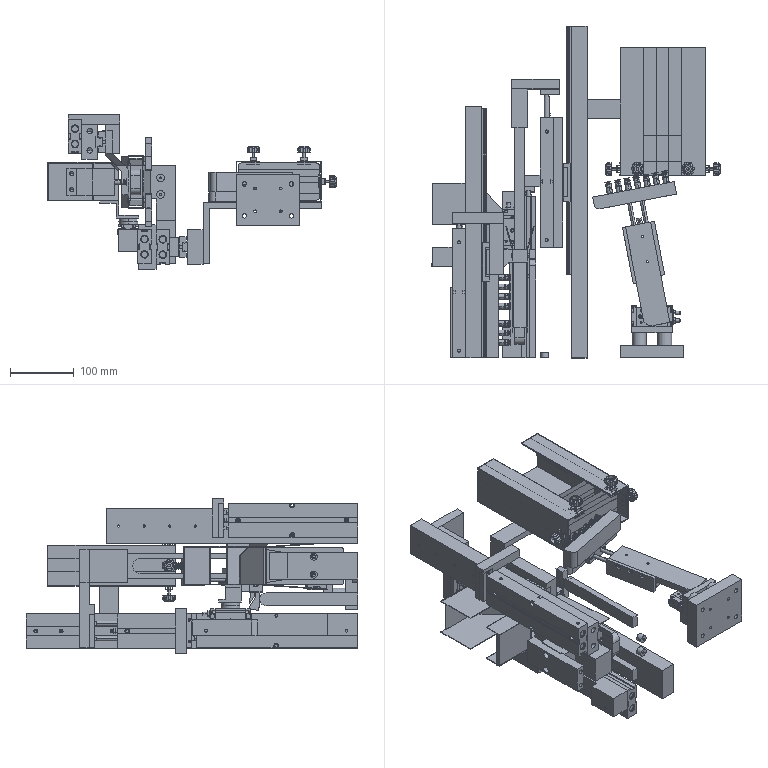Assembly | SolidWorks | mm | 91 component files | 107 solids | 3968 faces | box 451.44 x 520 x 242.54 mm | volume 3944049 mm3 | plane 1659 | cylinder 1465 | cone 700 | torus 144 | commonest cylinder face diameters 4.5 x136 6 x130 0.4 x90 8 x81 2.459 x80 4 x79 4.2 x70 3.5 x64
Bill of materials:
Counterweight | 2 |  | Rectangular prismatic block with a narrow slit running in from one top corner. The slit starts at an angle, turns straight along the length, and ends in a circular relief hole. A small cross hole goes through an adjacent face.
CylinderBracket2 | 1 |  | Rectangular bar with a shallow rectangular recess across part of one long face. It has two through holes in the large face and two drilled holes in one end face.
CylinderFixingBlockS | 1 |  | Rectangular block with a small rectangular tab sticking out from one face at about mid-height. There are two holes on each of two adjacent faces.
FeedBarrelPistonBracket2 | 1 |  | Long rectangular bar with a rectangular groove running the full length of one side face. A row of ten small holes runs along the groove, and the end face has two larger drilled holes.
FixedColumn | 1 |  | Plain long rectangular bar with no visible holes, slots or chamfers.
FunnelRotaryCylinderFixingPost | 1 |  | Long rectangular bar with a step in height along its length. It has a shallow recess with a rounded corner on one face and three small holes in a side face.
IAF11-H16-L390Slider | 2 |  | Rectangular block whose end profile is C-shaped, with chamfered outer corners and a central channel. The channel has rounded, shaped grooves near its inner corners. The top face has four holes, there are thin lengthwise lines, and the end sections are slightly larger than the main body.
IAF11-H16-L390SlideRail | 2 |  | Long, slender bar with a roughly rectangular cross-section, chamfered corners and shaped grooves on two opposite sides. It has a row of ten holes along its length.
InnerBagFunnel | 1 |  | Prismatic body with a U-shaped cutout, angled faces of about 45 degrees on one side, and a rectangular opening. It looks like separate stepped sections.
LargeFunnelFixing | 1 |  | Z-shaped plate of even thickness: two parallel flanges at different heights joined by an upright web. One round through hole is in the lower flange.
LimitRod | 2 |  | Thin plate with a tapering arm that ends in a rounded tip, joined to a wider rectangular end with two through holes. The plate is bent along a line near the wide end.
OuterBagExpansionSheetMetal | 2 |  | Rectangular bar with one end fully rounded (semicircular in one view) and the other end square.
OuterBagExpansionSheetMetalSidePlate | 2 |  | Thin flat rectangular strip with a solid cylindrical rod joined along one short edge; the rod is longer than the strip is wide and sticks out past both sides.
OuterBagExpansionSheetMetalSideSeal | 2 |  | Plain thin rectangular plate with sharp corners and no holes or other features that can be seen.
Copy_of_Part1 | 5 |  | Solid plain cylinder (rod or pin shape), several times longer than its diameter, with flat ends.
Copy_of_Part22 | 1 |  | L-shaped bar of rectangular cross-section: a long horizontal leg with a shorter leg bent or joined at 90 degrees at one end.
CopyOfOuterBagBox | 1 |  | Thin-walled rectangular hollow channel or box section, open at both ends, with a rectangular slot in the top wall that is open at one end. Small tab features stick out at one end on each wall.
PackagingBagLength | 2 |  | Very thin rectangular sheet with rounded corners.
PackagingBagShort | 1 |  | Very thin rectangular sheet with sharp corners.
ThumbNut | 5 | 45# Steel | Short cylindrical body with eight evenly spaced rounded lobes and grooves around the outside, chamfered top and bottom edges, and a central bore.
OuterBandCylinderFixingPlate | 1 |  | Long flat plate with one rounded corner, a stepped notch on one long edge, two small through holes, and a thicker raised or lower section along part of its length.
RotaryCylinderBase | 1 |  | Thick rectangular plate or block with eight through holes: four larger holes near the corners and four smaller holes in an inner rectangular pattern.
RotaryCylinderSupport | 1 |  | Rectangular plate with a stepped (L-shaped) profile along one edge and six through holes: four larger holes near the corners and two smaller holes in a middle row.
RotaryCylinderSupportPost | 4 |  | Thick-walled hollow cylinder (sleeve shape) with a central through bore; its length is about equal to its outside diameter.
RubberBufferPad | 2 |  | Short solid cylinder with a single small concentric through-bore; plain spacer/bushing-like shape.
Slider | 1 |  | Bracket made of a rectangular plate with four holes, a short angled transition section, and an offset rectangular leg. Gives a joggled/Z-shaped profile in side view.
SlideRailFixingPlate | 1 |  | Plain rectangular bar/prism, long and slender, with no visible holes or features.
SlidingAccessory | 1 |  | Rectangular-section frame bent into an L/U-like open shape with stepped ends. Four small holes on one outer face and two holes on another face.
SmallSuctionNozzle | 14 |  | Axisymmetric part with a cylindrical body, a reduced-diameter neck, and a flared conical cup at one end. Has a small central axial hole inside the cup.
SuctionCupConnector1 | 14 | 6061-T6 Aluminum | Stepped axisymmetric shaft/bushing with a central through-bore. It has a large center body with flat(s) cut on it, a smaller cylindrical end on one side, and a neck with a collar on the other.
SuctionCupMountingBlock(Fixed) | 1 |  | Rectangular block with a row of cross holes on one long face and two additional holes offset above and below the row center. A shallow raised step runs across the top/back face.
SuctionCupMountingBlock2 | 1 |  | Elongated rectangular bar with a stepped (rabbeted) cross-section and one rounded end. It has two small holes along one side and a larger hole in the end face.
SuctionCupMountingQuickConnector | 1 |  | Rectangular block with two parallel round through-holes in one face and stepped/notched edges along two opposite sides.
TelescopicRod | 1 |  | Long thin flat bar with a long obround through-slot and a thicker rectangular block at one end. The opposite end is rounded.
TelescopicRodFixingBlock | 1 |  | Flat plate shaped like an inverted L/J, with a wide upper section and a narrower stepped lower leg. Two small holes near the bottom of the leg.
WGN71-16-150-0CylinderBlock1 | 2 |  | Long rectangular bar assembly-like body: two stacked rectangular sections separated by a lengthwise groove, with T-slot-like notches in the cross-section. It has several round holes on faces and ends and a small stud protruding at one end.
WGN71-16-150-0PushRod1 | 2 |  | Two long, parallel cylindrical rods of equal length sticking out from one face of a narrow rectangular end block. The rods have plain round ends.
WGN71-16-200-0CylinderBlock | 1 |  | Long rectangular bar with T-slots running its full length on several faces, round holes on its faces, and short notches across the bar at mid-length.
WGN71-16-200-0PushRod | 1 |  | Two long, parallel cylindrical rods of equal length sticking out from one face of a narrow rectangular end block. The rods have plain round ends.
WGP01-2-R-M-0 | 2 |  | Compact rectangular housing with a raised round flanged disc on top. The disc has a ring of holes around a central recess. Two threaded-looking studs with hex nuts stick out from one end.
WGW01-10-30-0MainBody | 1 |  | Rectangular block with a plain top face that has two through-holes, two slots running along the underside, round holes in the side faces, and a small hex-headed stub at one end.
WGW01-10-30-0PushRod | 1 |  | Rectangular bar block with two parallel cylindrical pins sticking out at right angles from one face. The block has holes near each end.
Mates:
1. coincident | SuctionCupMountingBlock(Fixed)-1 face at (-606.696, -9.651, 394.468) dir (-1, 0, 0) | SuctionCupMountingQuickConnector-1 face at (-606.696, -53.651, 394.468) dir (1, 0, 0)
2. coincident | SuctionCupMountingBlock(Fixed)-1 face at (-571.465, -18.387, 352.468) dir (0, 0, -1) | SuctionCupMountingQuickConnector-1 face at (-571.465, 2.005, 352.468) dir (0, 0, -1)
3. parallel | SuctionCupMountingBlock(Fixed)-1 face at (-571.696, -9.651, 394.468) dir (1, 0, 0) | PackagingBagLength-2 face at (-546.806, -61.773, 373.468) dir (-1, 0, 0)
4. concentric | SmallSuctionNozzle-1 face at (-555.696, -21.651, 373.468) dir (-1, 0, 0) r 4.5 | SuctionCupConnector1-1 face at (-561.696, -21.651, 373.468) dir (-1, 0, 0) r 4.5
5. coincident | SmallSuctionNozzle-1 face at (-561.696, -21.651, 373.468) dir (-1, 0, 0) | SuctionCupConnector1-1 face at (-561.696, -21.651, 373.468) dir (1, 0, 0)
6. concentric | SuctionCupMountingBlock(Fixed)-1 face at (-585.696, -21.651, 373.468) dir (1, 0, 0) r 3 | SuctionCupConnector1-1 face at (-577.696, -21.651, 373.468) dir (1, 0, 0) r 3
7. coincident | SuctionCupMountingBlock(Fixed)-1 face at (-571.696, -9.651, 394.468) dir (1, 0, 0) | SuctionCupConnector1-1 face at (-571.696, -21.651, 373.468) dir (-1, 0, 0)
8. coincident | SuctionCupMountingBlock(Fixed)-1 face at (-604.696, -58.651, 394.468) dir (0, -1, 0) | SuctionCupMountingQuickConnector-1 face at (-571.465, -58.651, 394.468) dir (0, 1, 0)
9. concentric | WGW01-10-30-0PushRod-1 face at (-359.144, 54.528, 352.468) dir (-0.1885, 0.9821, 0) r 3 | WGW01-10-30-0MainBody-1 face at (-360.203, 60.042, 352.468) dir (0.1885, -0.9821, 0) r 3.1
10. concentric | WGW01-10-30-0PushRod-1 face at (-339.503, 58.299, 352.468) dir (-0.1885, 0.9821, 0) r 3 | WGW01-10-30-0MainBody-1 face at (-340.561, 63.813, 352.468) dir (0.1885, -0.9821, 0) r 3.1
11. distance | WGW01-10-30-0MainBody-1 face at (-352.079, 70.766, 349.468) dir (-0.1885, 0.9821, 0) | WGW01-10-30-0PushRod-1 face at (-357.053, 96.678, 358.468) dir (0.1885, -0.9821, 0)
12. coincident | OuterBandCylinderFixingPlate-1 face at (-331.696, -83.151, 359.468) dir (0, 0, -1) | WGW01-10-30-0MainBody-1 face at (-356.945, -25.885, 359.468) dir (0, 0, 1)
13. coincident | OuterBandCylinderFixingPlate-1 face at (-345.445, -85.791, 369.468) dir (-0.9821, -0.1885, 0) | WGW01-10-30-0MainBody-1 face at (-356.945, -25.885, 342.468) dir (-0.9821, -0.1885, 0)
14. coincident | OuterBandCylinderFixingPlate-1 face at (-359.22, 60.231, 369.468) dir (-0.1885, 0.9821, 0) | WGW01-10-30-0MainBody-1 face at (-350.382, 61.927, 359.468) dir (-0.1885, 0.9821, 0)
15. coincident | WGW01-10-30-0PushRod-1 face at (-378.658, 92.531, 358.468) dir (0, 0, 1) | SuctionCupMountingBlock2-1 face at (-420.887, 84.424, 358.468) dir (0, 0, -1)
16. coincident | WGW01-10-30-0PushRod-1 face at (-358.561, 104.535, 358.468) dir (-0.1885, 0.9821, 0) | SuctionCupMountingBlock2-1 face at (-422.396, 92.281, 388.468) dir (0.1885, -0.9821, 0)
17. concentric | WGP01-2-R-M-0-1 face at (-331.696, -83.151, 286.468) dir (0, 0, 1) r 14.5 | OuterBandCylinderFixingPlate-1 face at (-331.696, -83.151, 369.468) dir (0, 0, -1) r 14
18. coincident | WGP01-2-R-M-0-1 face at (-331.696, -97.151, 364.468) dir (0, 0, 1) | OuterBandCylinderFixingPlate-1 face at (-331.696, -83.151, 364.468) dir (0, 0, -1)
19. width | SuctionCupMountingBlock(Fixed)-1 face at (-571.465, -18.387, 394.468) dir (0, 0, 1) | SuctionCupMountingBlock(Fixed)-1 face at (-571.465, -18.387, 352.468) dir (0, 0, -1) | SuctionCupMountingBlock2-1 face at (-420.887, 84.424, 388.468) dir (0, 0, 1) | SuctionCupMountingBlock2-1 face at (-420.887, 84.424, 358.468) dir (0, 0, -1)
20. concentric | SuctionCupConnector1-19 face at (-311.225, 139.079, 373.468) dir (0.1885, -0.9821, 0) r 2.25 | SmallSuctionNozzle-19 face at (-311.696, 141.534, 373.468) dir (0.1885, -0.9821, 0) r 2.25
21. coincident | SuctionCupConnector1-19 face at (-310.659, 136.132, 373.468) dir (-0.1885, 0.9821, 0) | SmallSuctionNozzle-19 face at (-310.659, 136.132, 373.468) dir (0.1885, -0.9821, 0)
22. concentric | SuctionCupMountingBlock2-1 face at (-306.7, 115.509, 373.468) dir (-0.1885, 0.9821, 0) r 3 | SuctionCupConnector1-19 face at (-307.643, 120.419, 373.468) dir (-0.1885, 0.9821, 0) r 3
23. coincident | SuctionCupMountingBlock2-1 face at (-424.658, 104.066, 358.468) dir (-0.1885, 0.9821, 0) | SuctionCupConnector1-19 face at (-308.774, 126.312, 373.468) dir (0.1885, -0.9821, 0)
24. width | SuctionCupMountingBlock2-1 face at (-293.219, 108.933, 358.468) dir (0.9821, 0.1885, 0) | SuctionCupMountingBlock2-1 face at (-420.887, 84.424, 358.468) dir (-0.9821, -0.1885, 0) | WGW01-10-30-0PushRod-1 face at (-378.658, 92.531, 343.468) dir (-0.9821, -0.1885, 0) | WGW01-10-30-0PushRod-1 face at (-335.447, 100.826, 358.468) dir (0.9821, 0.1885, 0)
25. width | RotaryCylinderBase-1 face at (-381.696, -127.651, 305.468) dir (-1, 0, 0) | RotaryCylinderBase-1 face at (-281.696, -127.651, 305.468) dir (1, 0, 0) | RotaryCylinderSupport-1 face at (-363.696, -108.151, 371.718) dir (-1, 0, 0) | RotaryCylinderSupport-1 face at (-299.696, -108.151, 371.718) dir (1, 0, 0)
26. width | RotaryCylinderBase-1 face at (-381.696, -127.651, 305.468) dir (0, 0, -1) | RotaryCylinderBase-1 face at (-381.696, -127.651, 385.468) dir (0, 0, 1) | RotaryCylinderSupport-1 face at (-363.696, -108.151, 371.718) dir (0, 0, 1) | RotaryCylinderSupport-1 face at (-363.696, -108.151, 319.218) dir (0, 0, -1)
27. concentric | RotaryCylinderSupport-1 face at (-311.696, -93.151, 327.718) dir (0, 1, 0) r 2.75 | RotaryCylinderSupportPost-3 face at (-311.696, -108.151, 327.718) dir (0, -1, 0) r 3
28. coincident | RotaryCylinderSupport-1 face at (-331.696, -108.151, 336.468) dir (0, -1, 0) | RotaryCylinderSupportPost-3 face at (-311.696, -108.151, 327.718) dir (0, 1, 0)
29. distance | SuctionCupMountingBlock(Fixed)-1 face at (-571.696, -9.651, 394.468) dir (1, 0, 0) | RotaryCylinderBase-1 face at (-381.696, -127.651, 305.468) dir (-1, 0, 0)
30. coincident | RotaryCylinderBase-1 face at (-565.183, -127.651, -1.861) dir (0, 1, 0) | RotaryCylinderSupportPost-3 face at (-311.696, -127.651, 327.718) dir (0, -1, 0)
31. coincident | IAF11-H16-L390SlideRail-1 face at (-591.446, 242.349, 428.968) dir (1, 0, 0) | IAF11-H16-L390Slider-1 face at (-591.446, 362.376, 428.968) dir (-1, 0, 0)
32. width | IAF11-H16-L390Slider-1 face at (-586.446, 32.476, 452.168) dir (0, 0, 1) | IAF11-H16-L390Slider-1 face at (-592.246, 32.476, 420.168) dir (0, 0, -1) | IAF11-H16-L390SlideRail-1 face at (-601.146, 242.349, 428.668) dir (0, 0, -1) | IAF11-H16-L390SlideRail-1 face at (-595.963, 242.349, 443.668) dir (0, 0, 1)
33. width | FeedBarrelPistonBracket2-1 face at (-598.446, -147.651, 409.168) dir (0, 0, -1) | FeedBarrelPistonBracket2-1 face at (-598.446, -147.651, 463.168) dir (0, 0, 1) | IAF11-H16-L390SlideRail-1 face at (-595.963, 242.349, 443.668) dir (0, 0, 1) | IAF11-H16-L390SlideRail-1 face at (-601.146, 242.349, 428.668) dir (0, 0, -1)
34. coincident | FeedBarrelPistonBracket2-1 face at (-718.446, -147.651, 409.168) dir (0, -1, 0) | IAF11-H16-L390SlideRail-1 face at (-594.537, -147.651, 443.954) dir (0, -1, 0)
35. coincident | IAF11-H16-L390Slider-1 face at (-585.446, 32.476, 443.168) dir (1, 0, 0) | Slider-1 face at (-585.446, 3.436, 436.098) dir (-1, 0, 0)
36. width | IAF11-H16-L390Slider-1 face at (-585.446, 32.476, 436.168) dir (0, 1, 0) | IAF11-H16-L390Slider-1 face at (-585.446, -27.624, 436.168) dir (0, -1, 0) | Slider-1 face at (-550.446, -17.574, 453.668) dir (0, -1, 0) | Slider-1 face at (-550.446, 22.426, 453.668) dir (0, 1, 0)
37. concentric | Slider-1 face at (-550.446, 14.926, 423.668) dir (1, 0, 0) r 1.7 | IAF11-H16-L390Slider-1 face at (-585.446, 14.926, 423.668) dir (-1, 0, 0) r 1.23
38. coincident | Slider-1 face at (-550.446, 3.436, 436.098) dir (1, 0, 0) | OuterBagExpansionSheetMetal-1 face at (-550.446, -97.574, 373.468) dir (-1, 0, 0)
39. width | OuterBagExpansionSheetMetal-1 face at (-549.446, 22.426, 413.468) dir (0, 0, 1) | OuterBagExpansionSheetMetal-1 face at (-549.446, 22.426, 333.468) dir (0, 0, -1) | SuctionCupMountingBlock(Fixed)-1 face at (-571.465, -18.387, 352.468) dir (0, 0, -1) | SuctionCupMountingBlock(Fixed)-1 face at (-571.465, -18.387, 394.468) dir (0, 0, 1)
40. coincident | Slider-1 face at (-550.446, 22.426, 453.668) dir (0, 1, 0) | OuterBagExpansionSheetMetal-1 face at (-549.446, 22.426, 413.468) dir (0, 1, 0)
41. width | PackagingBagLength-2 face at (-546.581, 1.977, 402.718) dir (0, 0, 1) | PackagingBagLength-2 face at (-546.581, 1.977, 344.218) dir (0, 0, -1) | SuctionCupMountingBlock(Fixed)-1 face at (-571.465, -18.387, 394.468) dir (0, 0, 1) | SuctionCupMountingBlock(Fixed)-1 face at (-571.465, -18.387, 352.468) dir (0, 0, -1)
42. distance | OuterBagExpansionSheetMetal-1 face at (-549.446, -97.574, 373.468) dir (1, 0, 0) | OuterBagExpansionSheetMetal-2 face at (-527.446, -97.574, 373.468) dir (-1, 0, 0)
43. coincident | OuterBagExpansionSheetMetal-1 face at (-549.446, 22.426, 413.468) dir (0, 0, 1) | OuterBagExpansionSheetMetal-2 face at (-527.446, 22.426, 413.468) dir (0, 0, 1)
44. coincident | OuterBagExpansionSheetMetal-1 face at (-549.446, 22.426, 413.468) dir (0, 1, 0) | OuterBagExpansionSheetMetal-2 face at (-527.446, 22.426, 333.468) dir (0, 1, 0)
45. concentric | OuterBagExpansionSheetMetal-2 face at (-517.446, 12.426, 402.153) dir (-1, 0, 0) r 4 | OuterBagExpansionSheetMetalSidePlate-1 face at (-552.446, 12.426, 402.153) dir (1, 0, 0) r 3
46. distance | OuterBagExpansionSheetMetalSidePlate-1 face at (-548.446, -100.292, 409.517) dir (-1, 0, 0) | OuterBagExpansionSheetMetal-1 face at (-549.446, -97.574, 373.468) dir (1, 0, 0)
47. coincident | OuterBagExpansionSheetMetal-1 face at (-549.446, 22.426, 333.468) dir (0, 0, -1) | OuterBagExpansionSheetMetalSideSeal-2 face at (-550.446, 3.257, 333.468) dir (0, 0, 1)
48. coincident | OuterBagExpansionSheetMetal-2 face at (-526.446, -97.574, 373.468) dir (1, 0, 0) | OuterBagExpansionSheetMetalSideSeal-2 face at (-526.446, 22.426, 333.468) dir (1, 0, 0)
49. coincident | OuterBagExpansionSheetMetal-1 face at (-549.446, 22.426, 413.468) dir (0, 1, 0) | OuterBagExpansionSheetMetalSideSeal-2 face at (-550.446, 22.426, 333.468) dir (0, 1, 0)
50. concentric | OuterBagExpansionSheetMetalSidePlate-1 face at (-552.446, 12.426, 402.153) dir (1, 0, 0) r 3 | Counterweight-1 face at (-523.446, 12.426, 402.153) dir (1, 0, 0) r 3
51. coincident | OuterBagExpansionSheetMetalSidePlate-1 face at (-513.446, 12.426, 402.153) dir (1, 0, 0) | Counterweight-1 face at (-513.446, 26.616, 404.902) dir (1, 0, 0)
52. parallel | OuterBagExpansionSheetMetalSidePlate-1 face at (-530.636, 26.871, 401.647) dir (0, 0.0696, 0.9976) | Counterweight-1 face at (-523.446, 7.729, 442.578) dir (0, 0.0696, 0.9976)
53. concentric | WGN71-16-150-0CylinderBlock1-1 face at (-633.946, -142.651, 457.168) dir (0, -1, 0) r 4 | WGN71-16-150-0PushRod1-1 face at (-633.946, -138.074, 457.168) dir (0, 1, 0) r 4
54. concentric | WGN71-16-150-0CylinderBlock1-1 face at (-633.946, -142.651, 433.168) dir (0, -1, 0) r 4 | WGN71-16-150-0PushRod1-1 face at (-633.946, 69.926, 433.168) dir (0, -1, 0) r 4
55. distance | WGN71-16-150-0CylinderBlock1-1 face at (-631.446, 62.349, 445.168) dir (0, 1, 0) | WGN71-16-150-0PushRod1-1 face at (-633.946, 62.426, 418.668) dir (0, -1, 0)
56. coincident | FeedBarrelPistonBracket2-1 face at (-623.446, -147.651, 463.168) dir (-1, 0, 0) | WGN71-16-150-0CylinderBlock1-1 face at (-623.446, -147.651, 441.218) dir (1, 0, 0)
57. distance | FeedBarrelPistonBracket2-1 face at (-598.446, -147.651, 463.168) dir (0, 0, 1) | WGN71-16-150-0CylinderBlock1-1 face at (-644.446, -147.651, 472.168) dir (0, 0, 1)
58. coincident | Slider-1 face at (-550.446, -17.574, 453.668) dir (0, -1, 0) | SlidingAccessory-1 face at (-633.946, -17.574, 418.168) dir (0, -1, 0)
59. concentric | WGN71-16-200-0CylinderBlock-1 face at (-524.996, -142.651, 260.126) dir (0, -1, 0) r 4 | WGN71-16-200-0PushRod-1 face at (-524.996, -138.151, 260.126) dir (0, 1, 0) r 4
60. concentric | WGN71-16-200-0CylinderBlock-1 face at (-524.996, -142.651, 284.126) dir (0, -1, 0) r 4 | WGN71-16-200-0PushRod-1 face at (-524.996, 119.849, 284.126) dir (0, -1, 0) r 4
61. coincident | CylinderBracket2-1 face at (-633.696, -57.601, 395.168) dir (1, 0, 0) | SuctionCupMountingQuickConnector-1 face at (-633.696, 2.005, 394.468) dir (-1, 0, 0)
62. width | assembly face at (-743.489, 29.849, 340.126) dir (0, 0, -1) | assembly face at (-743.489, 29.849, 408.126) dir (0, 0, 1) | InnerBagFunnel-1 face at (-624.146, -40.37, 404.126) dir (0, 0, 1) | InnerBagFunnel-1 face at (-624.146, -40.37, 344.126) dir (0, 0, -1)
63. parallel | OuterBagExpansionSheetMetalSideSeal-2 face at (-550.446, 3.257, 332.468) dir (0, 0, -1) | WGP01-2-R-M-0-2 face at (-565.496, 28.112, 289.126) dir (0, 0, -1)
64. parallel | OuterBagExpansionSheetMetal-2 face at (-526.446, -97.574, 373.468) dir (1, 0, 0) | WGP01-2-R-M-0-2 face at (-535.496, 28.112, 289.126) dir (1, 0, 0)
65. concentric | WGP01-2-R-M-0-2 face at (-550.496, 52.112, 239.126) dir (0, 0, 1) r 2 | LargeFunnelFixing-1 face at (-550.496, 52.112, 296.126) dir (0, 0, 1) r 2.7
66. coincident | InnerBagFunnel-1 face at (-565.37, 60.55, 344.126) dir (0, 1, 0) | LargeFunnelFixing-1 face at (-624.146, 60.55, 354.126) dir (0, 1, 0)
67. coincident | InnerBagFunnel-1 face at (-595.37, 60.55, 414.126) dir (-1, 0, 0) | LargeFunnelFixing-1 face at (-595.37, 35.55, 344.126) dir (-1, 0, 0)
68. coincident | WGP01-2-R-M-0-2 face at (-536.496, 52.112, 317.126) dir (0, 0, 1) | LargeFunnelFixing-1 face at (-569.37, 35.55, 317.126) dir (0, 0, -1)
69. distance | WGN71-16-200-0CylinderBlock-1 face at (-527.496, 112.349, 272.126) dir (0, 1, 0) | WGN71-16-200-0PushRod-1 face at (-524.996, 112.349, 298.626) dir (0, -1, 0)
70. coincident | FunnelRotaryCylinderFixingPost-2 face at (-535.496, 112.349, 264.126) dir (1, 0, 0) | WGN71-16-200-0CylinderBlock-1 face at (-535.496, -147.651, 276.076) dir (-1, 0, 0)
71. concentric | assembly face at (-496.496, 410.483, 259.626) dir (0, 1, 0) r 4 | assembly face at (-496.496, 205.983, 259.626) dir (0, -1, 0) r 4
72. concentric | assembly face at (-496.496, 668.483, 283.626) dir (0, -1, 0) r 4 | assembly face at (-496.496, 205.983, 283.626) dir (0, -1, 0) r 4
73. distance | assembly face at (-498.996, 460.983, 271.626) dir (0, 1, 0) | assembly face at (-496.496, 660.983, 298.126) dir (0, -1, 0)
74. concentric | assembly face at (-1039.492, -117.162, 495.112) dir (0, -1, 0.002051) r 4 | assembly face at (-1039.492, 64.565, 494.739) dir (0, 1, -0.002051) r 4
75. concentric | assembly face at (-1039.492, -117.112, 519.112) dir (0, -1, 0.002051) r 4 | assembly face at (-1039.492, 322.613, 518.21) dir (0, -1, 0.002051) r 4
76. distance | assembly face at (-1041.992, 137.862, 506.589) dir (0, 1, -0.002051) | assembly face at (-1039.492, 315.143, 532.726) dir (0, -1, 0.002051)
77. concentric | Counterweight-3 face at (-513.446, 12.426, 344.782) dir (-1, 0, 0) r 3 | OuterBagExpansionSheetMetalSidePlate-2 face at (-552.446, 12.426, 344.782) dir (1, 0, 0) r 3
78. coincident | Counterweight-3 face at (-513.446, 26.617, 342.035) dir (1, 0, 0) | OuterBagExpansionSheetMetalSidePlate-2 face at (-513.446, 12.426, 344.782) dir (1, 0, 0)
79. coincident | Counterweight-1 face at (-513.446, 26.616, 404.902) dir (1, 0, 0) | Counterweight-3 face at (-513.446, 26.617, 342.035) dir (1, 0, 0)
80. concentric | OuterBagExpansionSheetMetal-2 face at (-517.446, 12.426, 344.782) dir (-1, 0, 0) r 4 | OuterBagExpansionSheetMetalSidePlate-2 face at (-552.446, 12.426, 344.782) dir (1, 0, 0) r 3
81. parallel | Counterweight-3 face at (-513.446, 19.211, 355.28) dir (0, -0.06975, 0.9976) | OuterBagExpansionSheetMetalSidePlate-2 face at (-530.636, 26.871, 345.29) dir (0, 0.06975, -0.9976)
82. coincident | FunnelRotaryCylinderFixingPost-2 face at (-550.496, 52.112, 299.126) dir (0, 0, 1) | WGN71-16-200-0CylinderBlock-1 face at (-535.496, -147.651, 299.126) dir (0, 0, 1)
83. angle | WGP01-2-R-M-0-2 face at (-537.196, 84.112, 302.126) dir (0, 1, 0) | LargeFunnelFixing-1 face at (-624.146, 70.55, 354.126) dir (0, 1, 0)
84. coincident | WGN71-16-200-0PushRod-1 face at (-534.996, 112.349, 298.626) dir (0, 0, 1) | assembly face at (-506.996, 200.983, 298.626) dir (0, 0, 1)
85. coincident | WGN71-16-200-0PushRod-1 face at (-534.996, 112.349, 245.626) dir (-1, 0, 0) | CylinderFixingBlockS-1 face at (-534.996, 120.349, 236.626) dir (-1, 0, 0)
86. concentric | assembly face at (-485.996, 328.983, 248.126) dir (-1, 0, 0) r 2.25 | CylinderFixingBlockS-1 face at (-506.996, 128.983, 248.126) dir (1, 0, 0) r 2.1
87. concentric | assembly face at (-506.996, 328.983, 295.126) dir (1, 0, 0) r 2.25 | CylinderFixingBlockS-1 face at (-506.996, 128.983, 295.126) dir (1, 0, 0) r 2.1
88. coincident | assembly face at (-506.996, 200.983, 275.576) dir (-1, 0, 0) | CylinderFixingBlockS-1 face at (-506.996, 120.349, 236.626) dir (1, 0, 0)
89. coincident | WGN71-16-200-0PushRod-1 face at (-524.996, 120.349, 298.626) dir (0, 1, 0) | CylinderFixingBlockS-1 face at (-534.996, 120.349, 236.626) dir (0, -1, 0)
90. coincident | assembly face at (-486.496, 660.983, 245.126) dir (0, 0, -1) | assembly face at (-506.496, 683.983, 245.126) dir (0, 0, -1)
91. coincident | assembly face at (-506.496, 660.983, 245.126) dir (-1, 0, 0) | assembly face at (-506.496, 683.983, 245.126) dir (-1, 0, 0)
92. coincident | assembly face at (-496.496, 668.983, 298.126) dir (0, 1, 0) | assembly face at (-496.496, 668.983, 298.626) dir (0, -1, 0)
93. concentric | assembly face at (-496.496, 230.983, 259.626) dir (0, -1, 0) r 4 | assembly face at (-496.496, 575.837, 259.626) dir (0, -1, 0) r 4
94. concentric | assembly face at (-496.496, 230.983, 283.626) dir (0, -1, 0) r 4 | assembly face at (-496.496, 367.837, 283.626) dir (0, 1, 0) r 4
95. distance | assembly face at (-493.996, 435.983, 271.626) dir (0, 1, 0) | assembly face at (-496.496, 568.337, 245.126) dir (0, -1, 0)
96. coincident | CylinderFixingBlockS-1 face at (-506.996, 120.349, 236.626) dir (1, 0, 0) | assembly face at (-506.996, 225.983, 244.626) dir (-1, 0, 0)
97. concentric | CylinderFixingBlockS-1 face at (-506.996, 128.983, 295.126) dir (1, 0, 0) r 2.1 | assembly face at (-506.996, 328.983, 295.126) dir (1, 0, 0) r 2.25
98. concentric | CylinderFixingBlockS-1 face at (-506.996, 128.983, 248.126) dir (1, 0, 0) r 2.1 | assembly face at (-485.996, 328.983, 248.126) dir (-1, 0, 0) r 2.25
99. concentric | WGN71-16-200-0PushRod-1 face at (-524.996, 112.349, 248.626) dir (0, 1, 0) r 1.621 | CylinderFixingBlockS-1 face at (-524.996, 120.349, 248.626) dir (0, -1, 0) r 1.65
100. coincident | assembly face at (-486.496, 591.337, 245.126) dir (1, 0, 0) | assembly face at (-486.496, 568.337, 298.126) dir (1, 0, 0)
101. coincident | assembly face at (-516.496, 591.337, 245.126) dir (0, 0, -1) | assembly face at (-486.496, 568.337, 245.126) dir (0, 0, -1)
102. coincident | assembly face at (-506.496, 576.337, 298.626) dir (0, -1, 0) | assembly face at (-496.496, 576.337, 245.126) dir (0, 1, 0)
103. concentric | WGN71-16-150-0CylinderBlock1-3 face at (-496.496, 30.983, 259.626) dir (0, -1, 0) r 4 | WGN71-16-150-0PushRod1-3 face at (-496.496, 272.996, 259.626) dir (0, -1, 0) r 4
104. concentric | WGN71-16-150-0CylinderBlock1-3 face at (-496.496, 30.983, 283.626) dir (0, -1, 0) r 4 | WGN71-16-150-0PushRod1-3 face at (-496.496, 64.996, 283.626) dir (0, 1, 0) r 4
105. distance | WGN71-16-150-0CylinderBlock1-3 face at (-493.996, 235.983, 271.626) dir (0, 1, 0) | WGN71-16-150-0PushRod1-3 face at (-496.496, 265.496, 245.126) dir (0, -1, 0)
106. coincident | CylinderFixingBlockS-1 face at (-506.996, 120.349, 236.626) dir (1, 0, 0) | WGN71-16-150-0CylinderBlock1-3 face at (-506.996, 25.983, 275.576) dir (-1, 0, 0)
107. concentric | CylinderFixingBlockS-1 face at (-506.996, 128.983, 248.126) dir (1, 0, 0) r 2.1 | WGN71-16-150-0CylinderBlock1-3 face at (-485.996, 128.983, 248.126) dir (-1, 0, 0) r 2.25
108. concentric | CylinderFixingBlockS-1 face at (-506.996, 128.983, 295.126) dir (1, 0, 0) r 2.1 | WGN71-16-150-0CylinderBlock1-3 face at (-506.996, 128.983, 295.126) dir (1, 0, 0) r 2.25
109. width | IAF11-H16-L390Slider-2 face at (-470.296, 157.533, 255.626) dir (0, 0, -1) | IAF11-H16-L390Slider-2 face at (-464.496, 157.533, 287.626) dir (0, 0, 1) | IAF11-H16-L390SlideRail-2 face at (-455.596, 372.349, 279.126) dir (0, 0, 1) | IAF11-H16-L390SlideRail-2 face at (-460.779, 372.349, 264.126) dir (0, 0, -1)
110. coincident | IAF11-H16-L390Slider-2 face at (-465.296, 487.433, 278.826) dir (1, 0, 0) | IAF11-H16-L390SlideRail-2 face at (-465.296, 372.349, 278.826) dir (-1, 0, 0)
111. coincident | FixedColumn-1 face at (-455.296, -147.651, -0.2817) dir (-1, 0, 0) | IAF11-H16-L390SlideRail-2 face at (-455.296, 372.349, 264.426) dir (1, 0, 0)
112. coincident | FixedColumn-1 face at (-455.296, 372.349, 264.126) dir (0, 0, 1) | IAF11-H16-L390SlideRail-2 face at (-460.779, 372.349, 264.126) dir (0, 0, -1)
113. coincident | FixedColumn-1 face at (-542.171, 372.349, -0.2817) dir (0, 1, 0) | IAF11-H16-L390SlideRail-2 face at (-462.205, 372.349, 263.839) dir (0, 1, 0)
114. coincident | WGN71-16-150-0CylinderBlock1-3 face at (-485.996, 25.983, 244.626) dir (0, 0, -1) | FixedColumn-1 face at (-458.296, 372.349, 244.626) dir (0, 0, -1)
115. width | WGN71-16-150-0CylinderBlock1-3 face at (-485.996, 25.983, 244.626) dir (0, 0, -1) | WGN71-16-150-0CylinderBlock1-3 face at (-506.996, 25.983, 298.626) dir (0, 0, 1) | SlideRailFixingPlate-1 face at (-471.296, 25.983, 286.626) dir (0, 0, 1) | SlideRailFixingPlate-1 face at (-471.296, 25.983, 256.626) dir (0, 0, -1)
116. coincident | WGN71-16-150-0CylinderBlock1-3 face at (-486.196, 228.983, 275.576) dir (0, 1, 0) | SlideRailFixingPlate-1 face at (-235.297, 228.983, 271.626) dir (0, 1, 0)
117. width | SlideRailFixingPlate-1 face at (-235.297, 25.983, 271.626) dir (0, -1, 0) | SlideRailFixingPlate-1 face at (-235.297, 228.983, 271.626) dir (0, 1, 0) | IAF11-H16-L390Slider-2 face at (-471.296, 157.533, 271.626) dir (0, 1, 0) | IAF11-H16-L390Slider-2 face at (-471.296, 97.433, 271.626) dir (0, -1, 0)
118. coincident | FixedColumn-1 face at (-433.296, 372.349, 298.626) dir (1, 0, 0) | OuterBagStorageAssembly-1/Copy_of_Part22-1 face at (-433.296, 227.349, 245.168) dir (-1, 0, 0)
119. distance | FixedColumn-1 face at (-542.171, 372.349, -0.2817) dir (0, 1, 0) | OuterBagStorageAssembly-1/Copy_of_Part22-1 face at (-315.175, 257.349, 386.24) dir (0, 1, 0)
120. concentric | SuctionCupMountingBlock(Fixed)-1 face at (-585.696, -93.651, 373.468) dir (1, 0, 0) r 3 | SuctionCupConnector1-26 face at (-577.696, -93.651, 373.468) dir (1, 0, 0) r 3
121. coincident | SuctionCupMountingBlock(Fixed)-1 face at (-571.696, -9.651, 394.468) dir (1, 0, 0) | SuctionCupConnector1-26 face at (-571.696, -93.651, 373.468) dir (-1, 0, 0)
122. concentric | SuctionCupConnector1-26 face at (-561.696, -93.651, 373.468) dir (-1, 0, 0) r 4.5 | SmallSuctionNozzle-26 face at (-555.696, -93.651, 373.468) dir (-1, 0, 0) r 4.5
123. coincident | SuctionCupConnector1-26 face at (-556.196, -93.651, 373.468) dir (1, 0, 0) | SmallSuctionNozzle-26 face at (-556.196, -93.651, 373.468) dir (-1, 0, 0)
124. coincident | LimitRod-1 face at (-513.446, -3.651, 321.371) dir (1, 0, 0) | LimitRod-2 face at (-513.446, -3.651, 423.196) dir (1, 0, 0)
125. coincident | Counterweight-1 face at (-513.446, 26.616, 404.902) dir (1, 0, 0) | LimitRod-2 face at (-513.446, -3.651, 423.196) dir (1, 0, 0)
126. parallel | PackagingBagShort-1 face at (-26.336, 10.383, 140.943) dir (0, 0, -1) | PackagingBagLength-1 face at (-26.336, 10.383, 181.748) dir (0, 0, -1)
127. distance | PackagingBagShort-1 face at (1.264, -44.767, 141.168) dir (1, 0, 0) | PackagingBagLength-1 face at (2.914, 74.133, 181.973) dir (1, 0, 0)
128. distance | PackagingBagShort-1 face at (1.264, -44.767, 141.168) dir (0, -1, 0) | PackagingBagLength-1 face at (-55.586, -53.367, 181.973) dir (0, -1, 0)
129. width | CopyOfOuterBagBox-1 face at (5.664, 76.883, 203.221) dir (0, 1, 0) | CopyOfOuterBagBox-1 face at (5.664, -56.117, 203.221) dir (0, -1, 0) | PackagingBagLength-1 face at (-55.586, 74.133, 181.973) dir (0, 1, 0) | PackagingBagLength-1 face at (-55.586, -53.367, 181.973) dir (0, -1, 0)
130. width | CopyOfOuterBagBox-1 face at (-58.336, 76.883, 203.221) dir (-1, 0, 0) | CopyOfOuterBagBox-1 face at (5.664, 76.883, 203.221) dir (1, 0, 0) | PackagingBagLength-1 face at (2.914, 74.133, 181.973) dir (1, 0, 0) | PackagingBagLength-1 face at (-55.586, 74.133, 181.973) dir (-1, 0, 0)
131. coincident | CopyOfOuterBagBox-1 face at (5.664, 76.883, 203.221) dir (1, 0, 0) | Copy_of_Part22-1 face at (5.664, -108.117, 114.03) dir (-1, 0, 0)
132. concentric | ThumbNut-1 face at (-71.704, -29.117, 193.221) dir (1, 0, 0) r 2.1 | Copy_of_Part1-1 face at (-56.704, -29.117, 193.221) dir (-1, 0, 0) r 2.1
133. coincident | ThumbNut-1 face at (-76.704, -29.117, 193.221) dir (-1, 0, 0) | Copy_of_Part1-1 face at (-76.704, -29.117, 193.221) dir (-1, 0, 0)
134. concentric | Copy_of_Part1-2 face at (4.911, 9.883, 193.221) dir (1, 0, 0) r 2.1 | ThumbNut-2 face at (19.911, 9.883, 193.221) dir (-1, 0, 0) r 2.1
135. coincident | Copy_of_Part1-2 face at (24.911, 9.883, 193.221) dir (1, 0, 0) | ThumbNut-2 face at (24.911, 9.883, 193.221) dir (1, 0, 0)
136. concentric | CopyOfOuterBagBox-1 face at (11.664, 9.883, 193.221) dir (1, 0, 0) r 2.1 | Copy_of_Part1-2 face at (4.911, 9.883, 193.221) dir (1, 0, 0) r 2.1
137. concentric | Copy_of_Part1-3 face at (-26.336, -54.485, 193.221) dir (0, -1, 0) r 2.1 | ThumbNut-3 face at (-26.336, -69.485, 193.221) dir (0, 1, 0) r 2.1
138. coincident | Copy_of_Part1-3 face at (-26.336, -74.485, 193.221) dir (0, -1, 0) | ThumbNut-3 face at (-26.336, -74.485, 193.221) dir (0, -1, 0)
139. concentric | CopyOfOuterBagBox-1 face at (-26.336, -62.117, 193.221) dir (0, -1, 0) r 2.1 | Copy_of_Part1-3 face at (-26.336, -54.485, 193.221) dir (0, -1, 0) r 2.1
140. concentric | CopyOfOuterBagBox-1 face at (-58.336, -29.117, 193.221) dir (-1, 0, 0) r 2.1 | Copy_of_Part1-1 face at (-56.704, -29.117, 193.221) dir (-1, 0, 0) r 2.1
141. coincident | CopyOfOuterBagBox-1 face at (5.664, 76.883, 203.221) dir (0, 1, 0) | Copy_of_Part22-1 face at (5.664, 76.883, 114.03) dir (0, 1, 0)